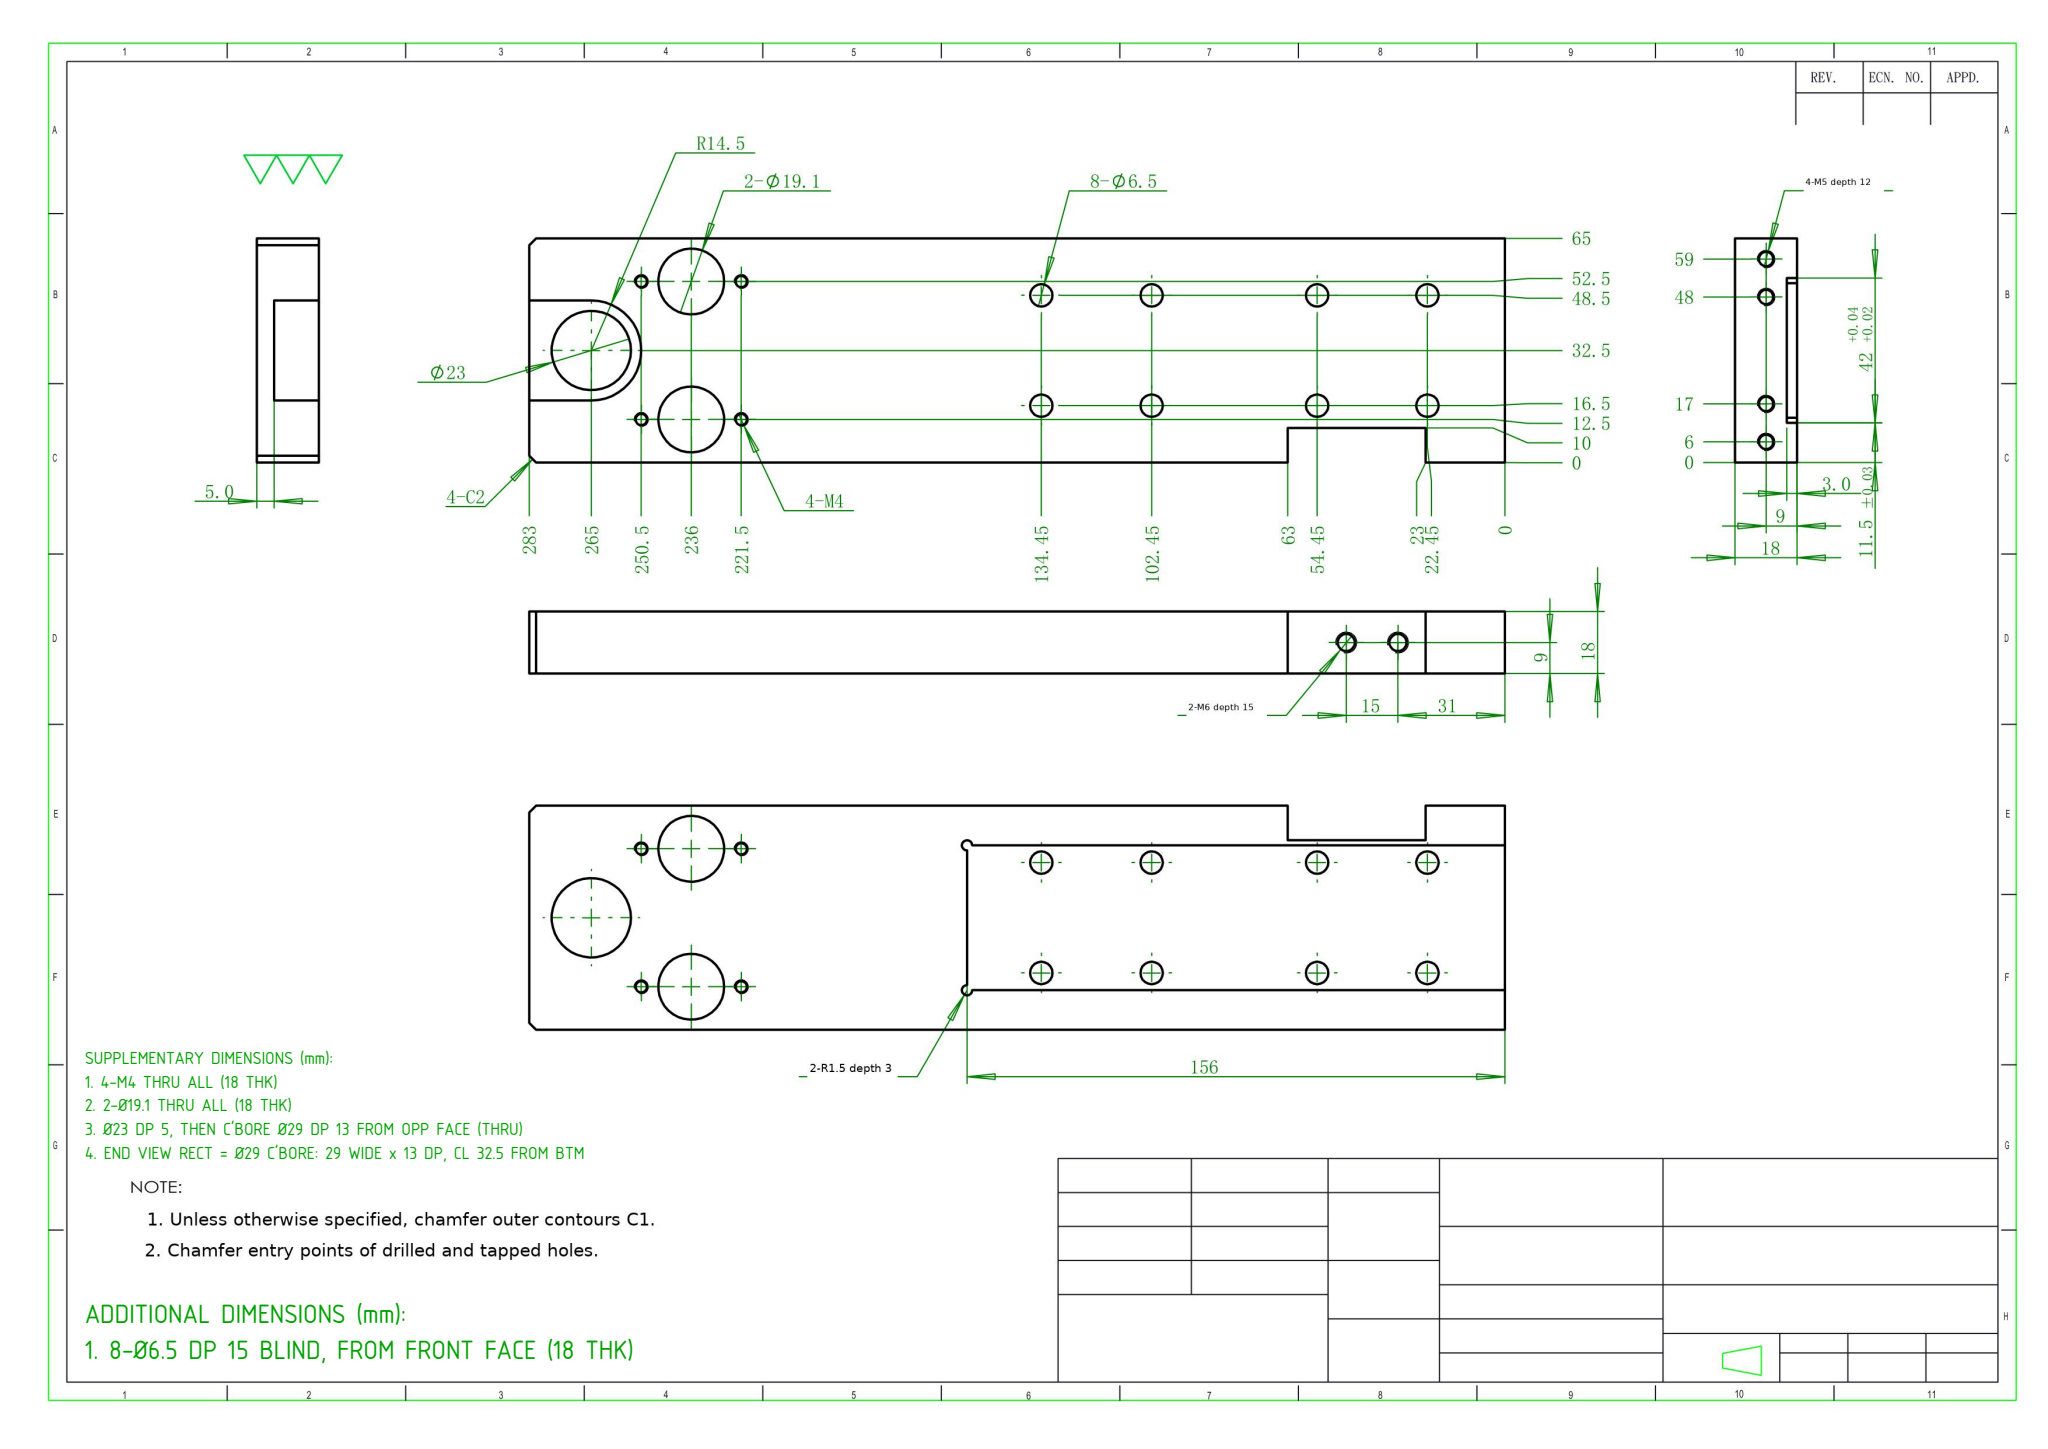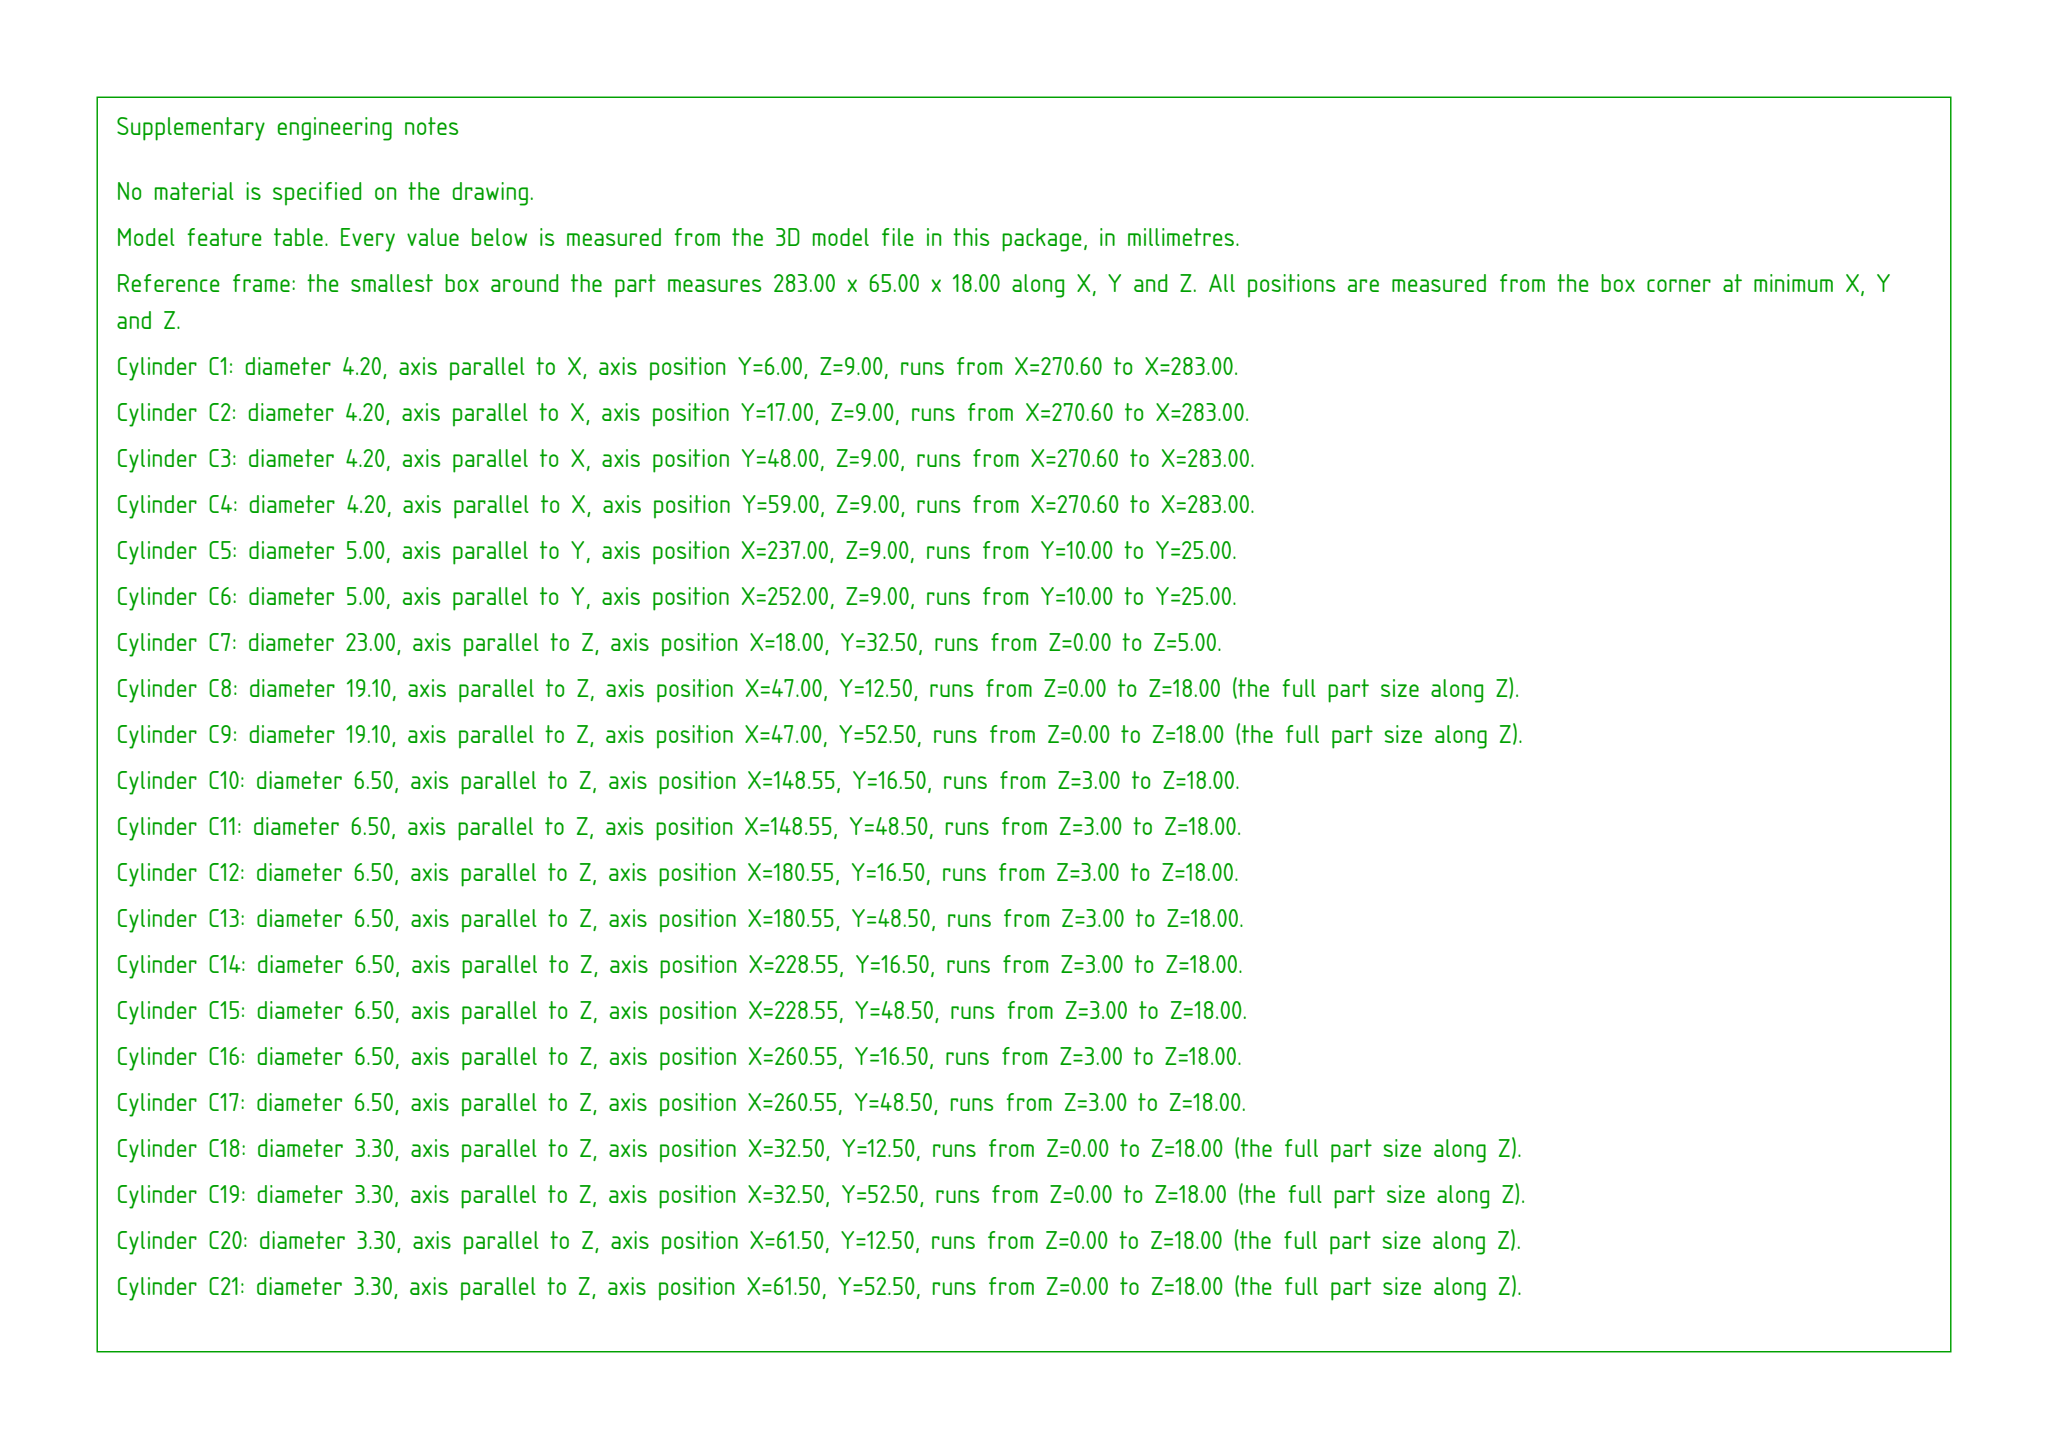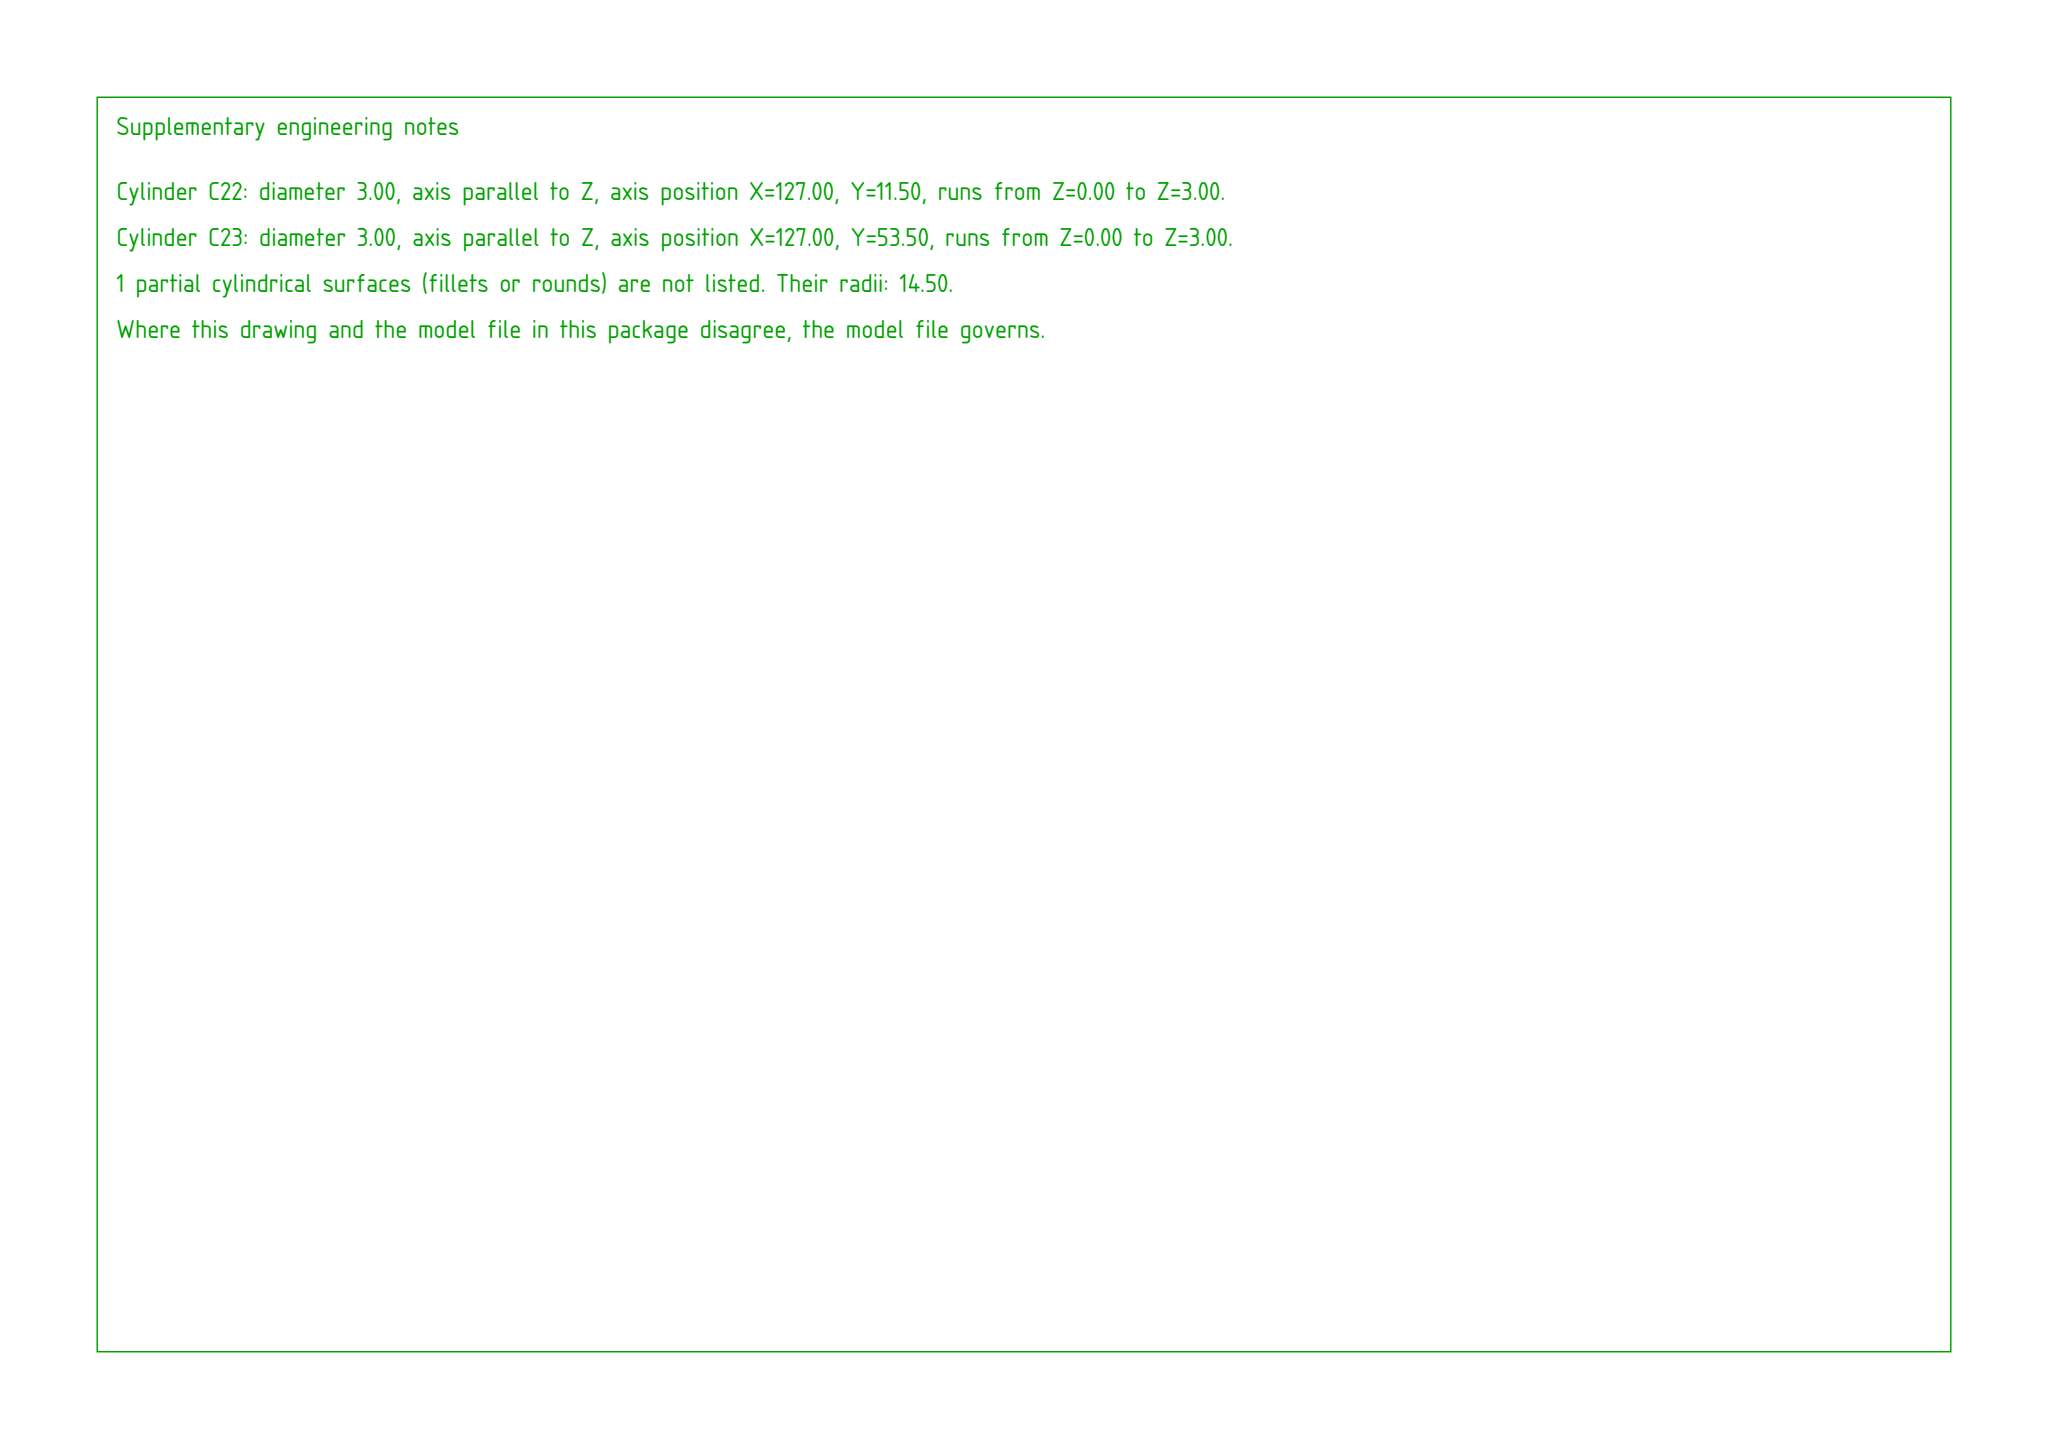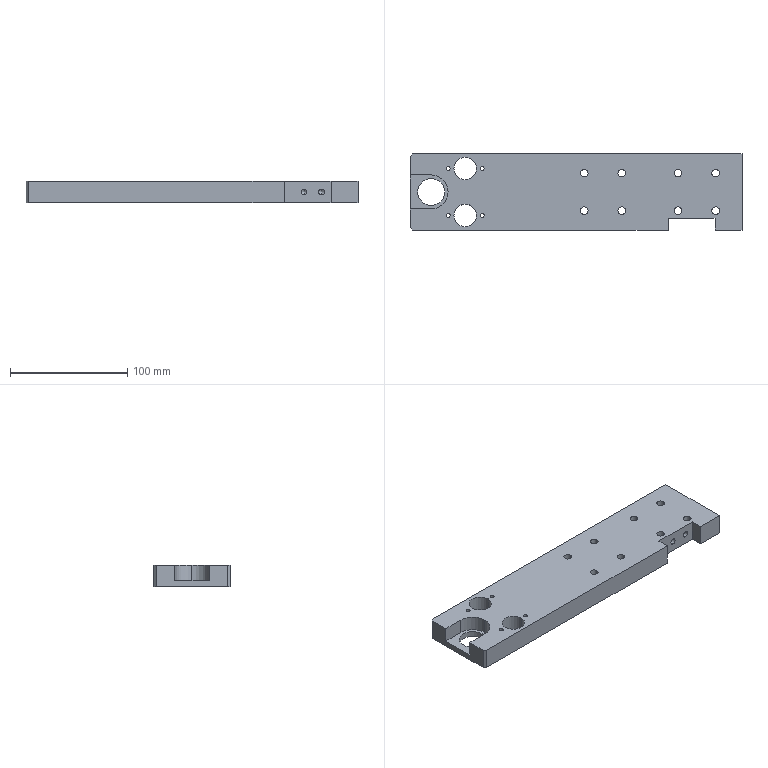Part | SolidWorks | mm | 1 solid | 79 faces | box 283 x 65 x 18 mm | volume 274762 mm3 | cylinder 48 | plane 19 | cone 12 | commonest cylinder face diameters 6.5 x16 3.3 x8 4.2 x8 3 x4 5 x4 19.1 x4 23 x2 29 x2
build123d program:
from build123d import *

# Parameters (mm, degrees)
SKETCH1_W                  = 300
SKETCH1_H                  = 65
BOSS_EXTRUDE1_DEPTH        = 18
SKETCH11_W                 = 3
SKETCH11_H                 = 42
CUT_EXTRUDE1_DEPTH         = 173
CUT_EXTRUDE2_DEPTH         = 155.532
CHAMFER1_SIZE              = 1
SKETCH18_R                 = 9.55
CUT_EXTRUDE3_DEPTH         = 155.532
CUT_EXTRUDE7_DEPTH         = 13
SKETCH23_R                 = 11.5
CUT_EXTRUDE8_DEPTH         = 155.03
SKETCH24_W                 = 40
SKETCH24_H                 = 10
CUT_EXTRUDE9_DEPTH         = 155.532
F_5_5_5_5_DIAMETER_HOLE1_D = 6.5
CHAMFER2_SIZE              = 2
M6_TAPPED_HOLE3_D          = 5
M6_TAPPED_HOLE3_DEPTH      = 15
M6_TAPPED_HOLE3_TIP        = 1.502
SKETCH31_W                 = 17
SKETCH31_H                 = 65
CUT_EXTRUDE10_DEPTH        = 155.532
M5_TAPPED_HOLE1_D          = 4.2
M5_TAPPED_HOLE1_DEPTH      = 12.4
M5_TAPPED_HOLE1_TIP        = 1.262
M4_TAPPED_HOLE1_D          = 3.3
SKETCH38_R                 = 1.5
CUT_EXTRUDE12_DEPTH        = 3


with BuildPart() as part:
    # Sketch1 → Boss-Extrude1 (new body)
    with BuildSketch(Plane.XY):
        Rectangle(SKETCH1_W, SKETCH1_H)
    extrude(amount=BOSS_EXTRUDE1_DEPTH)

    # Sketch11 → Cut-Extrude1 (cut)
    with BuildSketch(Plane(origin=(150, 0, 0), x_dir=(0, 0, -1), z_dir=(1, 0, 0))):
        with Locations((-1.5, 0)):
            Rectangle(SKETCH11_W, SKETCH11_H)
    extrude(amount=-CUT_EXTRUDE1_DEPTH, mode=Mode.SUBTRACT)

    # Sketch17 → Cut-Extrude2 (cut, through all)
    with BuildSketch(Plane.XY.offset(18)):
        Polygon((150, -5.5), (140, -5.5), (140, -10.5), (133, -10.5), (133, 10.5), (140, 10.5), (140, 5.5), (150, 5.5), align=None)
    extrude(amount=-CUT_EXTRUDE2_DEPTH, mode=Mode.SUBTRACT)

    # Chamfer1
    chamfer1_edges = [part.edges().sort_by_distance(p)[0] for p in [
        (150, 5.5, 10.5),
        (150, -5.5, 10.5),
        (140, -5.5, 10.5),
        (140, 5.5, 10.5),
    ]]
    chamfer(chamfer1_edges, length=CHAMFER1_SIZE)

    # Sketch18 → Cut-Extrude3 (cut, through all)
    with BuildSketch(Plane.XY.offset(18)):
        with Locations((-103, 20)):
            Circle(SKETCH18_R)
        with Locations(Location((-103, -20, 0), (0, 0, 180))):
            Circle(SKETCH18_R)
    extrude(amount=-CUT_EXTRUDE3_DEPTH, mode=Mode.SUBTRACT)

    # Sketch22 → Cut-Extrude7 (cut)
    with BuildSketch(Plane.XY.offset(18)):
        with BuildLine():
            Line((-150, 14.5), (-132, 14.5))
            ThreePointArc((-132, 14.5), (-117.5, 0), (-132, -14.5))
            Line((-132, -14.5), (-150, -14.5))
            ThreePointArc((-150, -14.5), (-164.5, 0), (-150, 14.5))
        make_face()
    extrude(amount=-CUT_EXTRUDE7_DEPTH, mode=Mode.SUBTRACT)

    # Sketch23 → Cut-Extrude8 (cut, through all)
    with BuildSketch(Plane.XY.offset(5)):
        with Locations((-132, 0)):
            Circle(SKETCH23_R)
    extrude(amount=-CUT_EXTRUDE8_DEPTH, mode=Mode.SUBTRACT)

    # Sketch24 → Cut-Extrude9 (cut, through all)
    with BuildSketch(Plane.XY.offset(18)):
        with Locations((90, -27.5)):
            Rectangle(SKETCH24_W, SKETCH24_H)
    extrude(amount=-CUT_EXTRUDE9_DEPTH, mode=Mode.SUBTRACT)

    # 5.5 _5.5_ Diameter Hole1 (through all)
    with Locations(Plane.XY.offset(18)):
        with Locations((-1.45, 16), (30.55, 16), (-1.45, -16), (30.55, -16), (78.55, 16), (110.55, 16), (110.55, -16), (78.55, -16)):
            Hole(F_5_5_5_5_DIAMETER_HOLE1_D / 2)

    # Chamfer2
    chamfer2_edges = [part.edges().sort_by_distance(p)[0] for p in [
        (150, -32.5, 9),
        (-150, -32.5, 9),
        (-150, 32.5, 9),
        (150, 32.5, 9),
    ]]
    chamfer(chamfer2_edges, length=CHAMFER2_SIZE)

    # M6 Tapped Hole3
    with Locations(Plane(origin=(0, -22.5, 0), x_dir=(-1, 0, 0), z_dir=(0, -1, 0))):
        with Locations((-87, -9), (-102, -9)):
            Hole(M6_TAPPED_HOLE3_D / 2, depth=M6_TAPPED_HOLE3_DEPTH)
            with Locations((0, 0, -(M6_TAPPED_HOLE3_DEPTH + M6_TAPPED_HOLE3_TIP / 2))):  # 118° drill point
                Cone(0, M6_TAPPED_HOLE3_D / 2, M6_TAPPED_HOLE3_TIP, mode=Mode.SUBTRACT)

    # Sketch31 → Cut-Extrude10 (cut, through all)
    with BuildSketch(Plane.XY.offset(18)):
        with Locations((141.5, 0)):
            Rectangle(SKETCH31_W, SKETCH31_H)
    extrude(amount=-CUT_EXTRUDE10_DEPTH, mode=Mode.SUBTRACT)

    # M5 Tapped Hole1
    with Locations(Plane(origin=(133, 0, 0), x_dir=(0, 0, -1), z_dir=(1, 0, 0))):
        with Locations((-9, -26.5), (-9, -15.5), (-9, 15.5), (-9, 26.5)):
            Hole(M5_TAPPED_HOLE1_D / 2, depth=M5_TAPPED_HOLE1_DEPTH)
            with Locations((0, 0, -(M5_TAPPED_HOLE1_DEPTH + M5_TAPPED_HOLE1_TIP / 2))):  # 118° drill point
                Cone(0, M5_TAPPED_HOLE1_D / 2, M5_TAPPED_HOLE1_TIP, mode=Mode.SUBTRACT)

    # M4 Tapped Hole1 (through all)
    with Locations(Plane.XY.offset(18)):
        with Locations((-88.5, -20), (-117.5, -20), (-88.5, 20), (-117.5, 20)):
            Hole(M4_TAPPED_HOLE1_D / 2)

    # Sketch38 → Cut-Extrude12 (cut)
    with BuildSketch(Plane(origin=(0, 0, 0), x_dir=(-1, 0, 0), z_dir=(0, 0, -1))):
        with Locations((23, 21)):
            Circle(SKETCH38_R)
        with Locations((23, -21)):
            Circle(SKETCH38_R)
    extrude(amount=-CUT_EXTRUDE12_DEPTH, mode=Mode.SUBTRACT)


solid = part.part